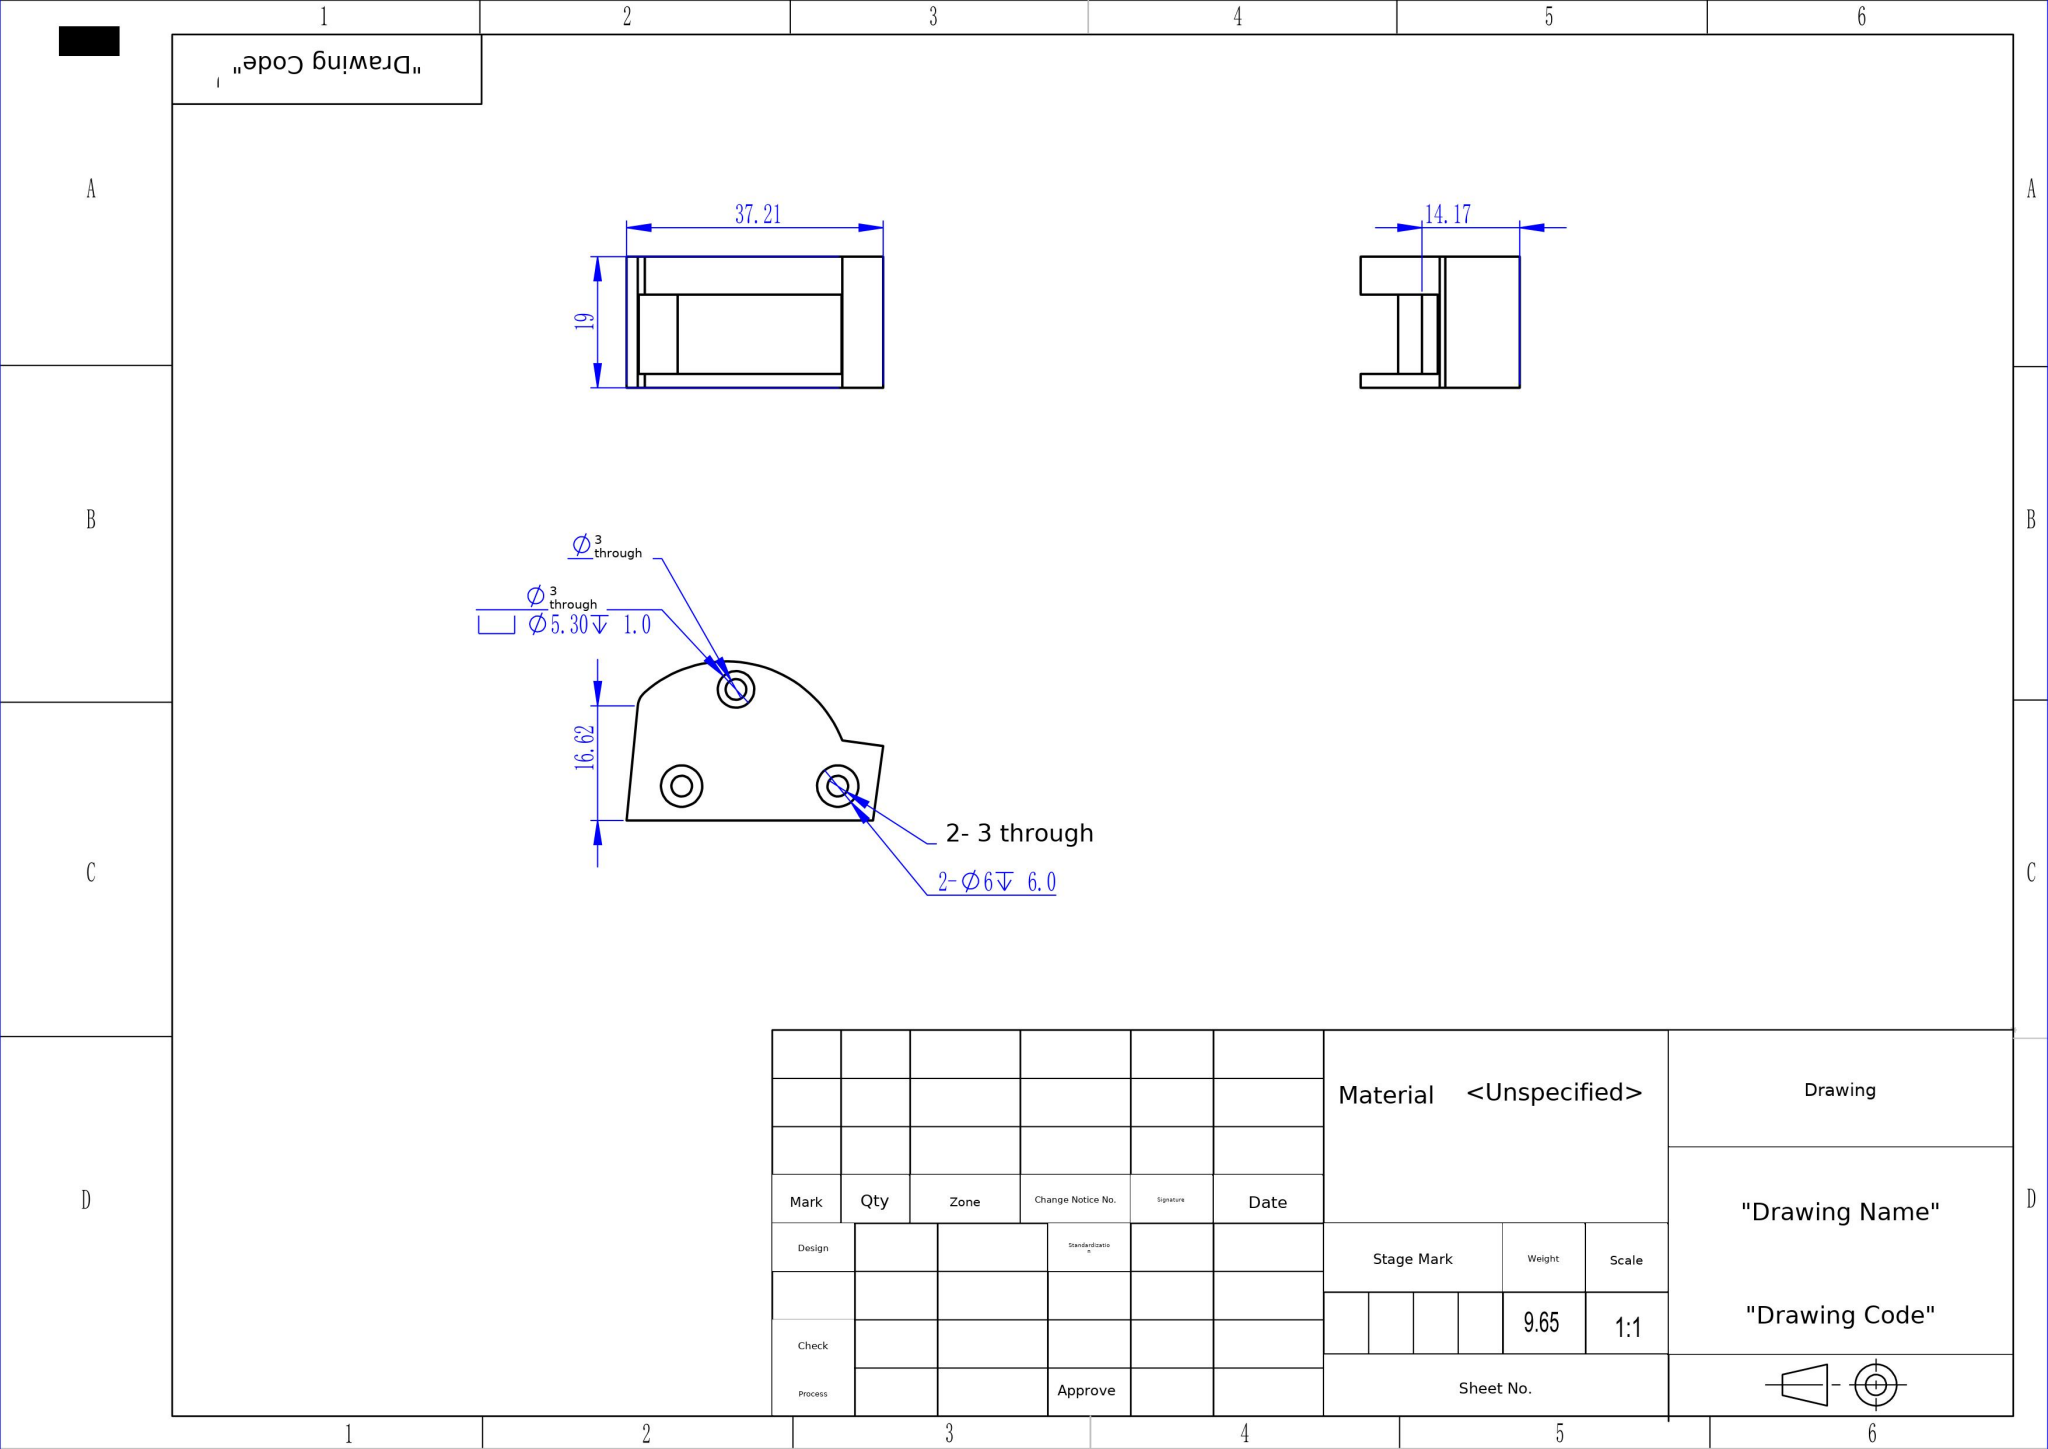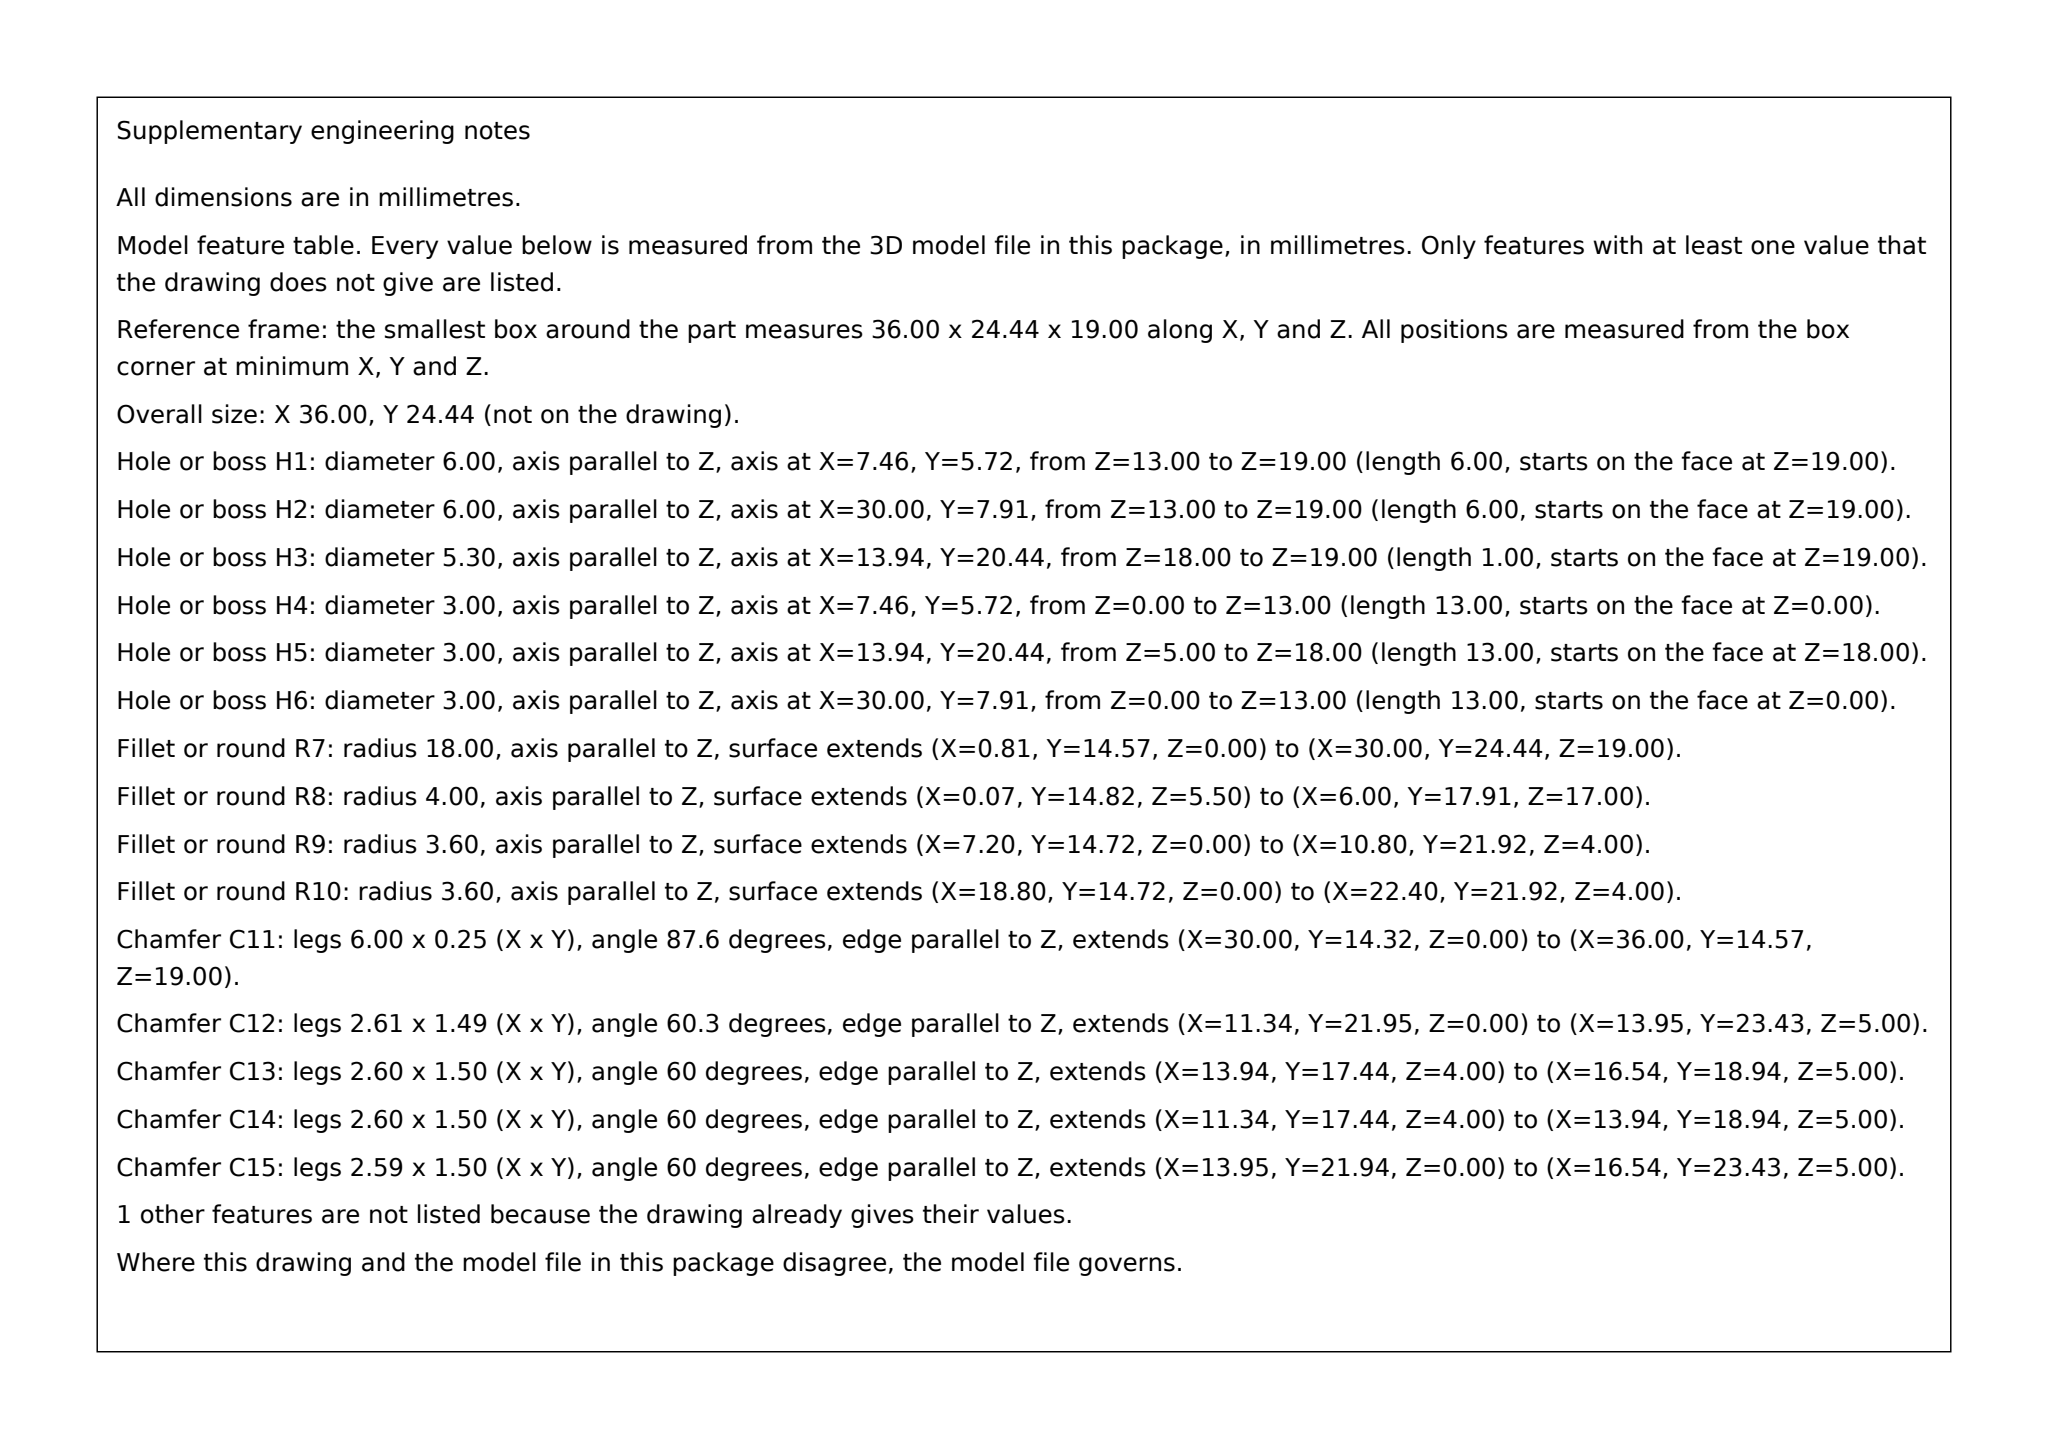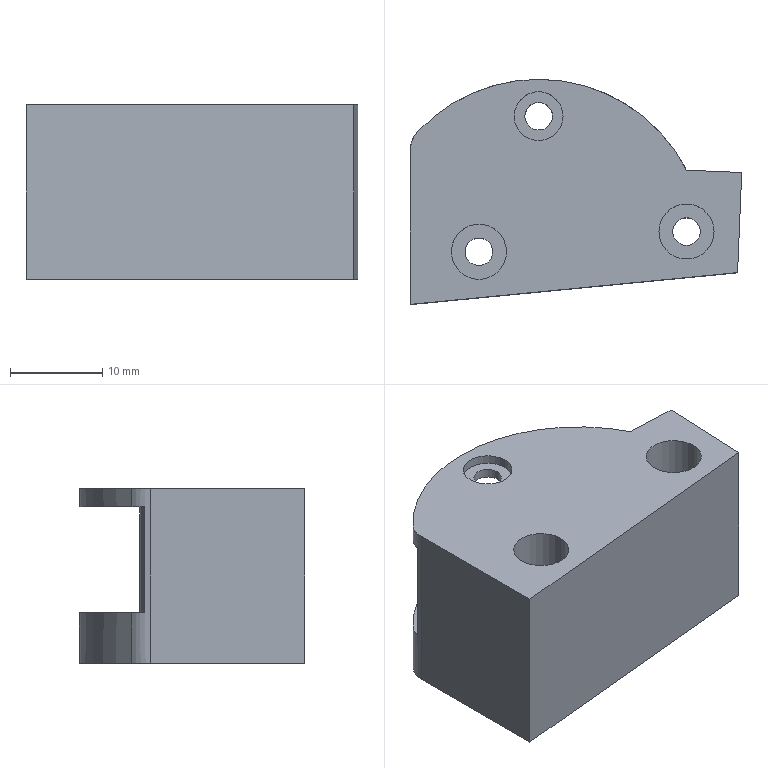Part | SolidWorks | mm | 1 solid | 43 faces | box 36 x 24.44 x 19 mm | volume 9651 mm3 | plane 23 | cylinder 20 | commonest cylinder face diameters 3 x8 6 x5 7.2 x3 5.3 x2 36 x1 8 x1